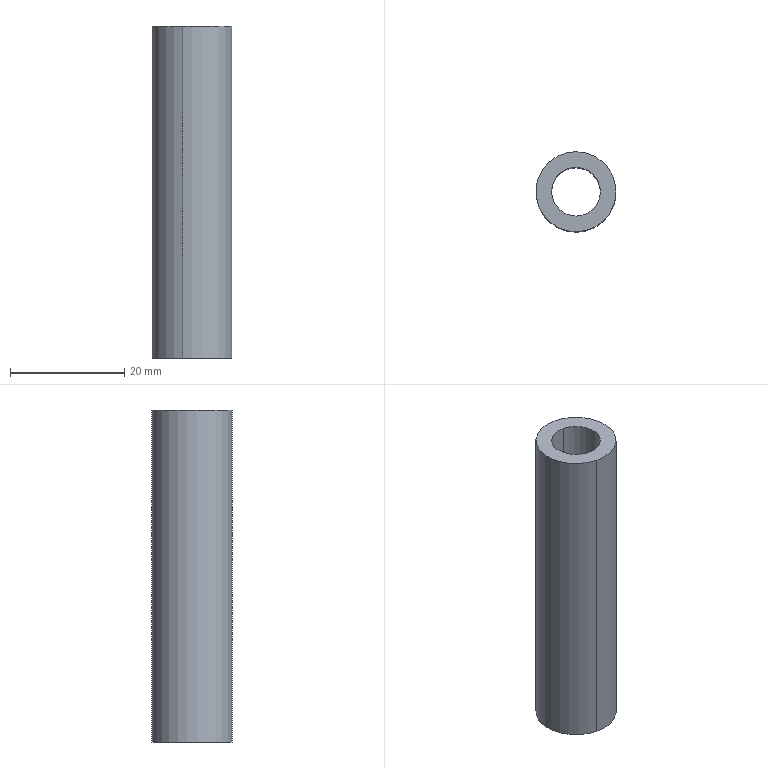Component | SolidWorks | JF21-110.2-20-1-SOLID1-1 | 1 solid | 6 faces | box 14 x 14 x 58 mm | volume 5637 mm3 | cylinder 4 | plane 2 | commonest cylinder face diameters 8.5 x2 14 x2
STEP:
#1=CARTESIAN_POINT('',(-0.03911,-0.1725,-10.984));
#2=VERTEX_POINT('',#1);
#3=CARTESIAN_POINT('',(0.03911,0.1528,-10.984));
#4=VERTEX_POINT('',#3);
#5=CARTESIAN_POINT('',(-0.,-0.009843,-10.984));
#6=DIRECTION('',(0.,-0.,1.));
#7=DIRECTION('',(0.2337,0.9723,0.));
#8=AXIS2_PLACEMENT_3D('',#5,#6,#7);
#9=CIRCLE('',#8,0.1673);
#10=EDGE_CURVE('',#2,#4,#9,.T.);
#11=ORIENTED_EDGE('',*,*,#10,.T.);
#12=CARTESIAN_POINT('',(0.03911,0.1528,-13.268));
#13=VERTEX_POINT('',#12);
#14=CARTESIAN_POINT('',(0.03911,0.1528,-10.984));
#15=DIRECTION('',(0.,-0.,1.));
#16=VECTOR('',#15,39.37);
#17=LINE('',#14,#16);
#18=EDGE_CURVE('',#13,#4,#17,.T.);
#19=ORIENTED_EDGE('',*,*,#18,.F.);
#20=CARTESIAN_POINT('',(-0.03911,-0.1725,-13.268));
#21=VERTEX_POINT('',#20);
#22=CARTESIAN_POINT('',(-0.,-0.009843,-13.268));
#23=DIRECTION('',(0.,-0.,1.));
#24=DIRECTION('',(0.2337,0.9723,0.));
#25=AXIS2_PLACEMENT_3D('',#22,#23,#24);
#26=CIRCLE('',#25,0.1673);
#27=EDGE_CURVE('',#21,#13,#26,.T.);
#28=ORIENTED_EDGE('',*,*,#27,.F.);
#29=CARTESIAN_POINT('',(-0.03911,-0.1725,-10.984));
#30=DIRECTION('',(0.,-0.,1.));
#31=VECTOR('',#30,39.37);
#32=LINE('',#29,#31);
#33=EDGE_CURVE('',#21,#2,#32,.T.);
#34=ORIENTED_EDGE('',*,*,#33,.T.);
#35=EDGE_LOOP('',(#11,#19,#28,#34));
#36=FACE_OUTER_BOUND('',#35,.T.);
#37=CARTESIAN_POINT('',(-0.,-0.009843,-10.984));
#38=DIRECTION('',(-0.,0.,-1.));
#39=DIRECTION('',(0.2337,0.9723,0.));
#40=AXIS2_PLACEMENT_3D('',#37,#38,#39);
#41=CYLINDRICAL_SURFACE('',#40,0.1673);
#42=ADVANCED_FACE('',(#36),#41,.F.);
#43=CARTESIAN_POINT('',(0.06441,0.2581,-10.984));
#44=VERTEX_POINT('',#43);
#45=CARTESIAN_POINT('',(-0.06441,-0.2778,-10.984));
#46=VERTEX_POINT('',#45);
#47=CARTESIAN_POINT('',(-0.,-0.009843,-10.984));
#48=DIRECTION('',(0.,-0.,1.));
#49=DIRECTION('',(0.2337,0.9723,0.));
#50=AXIS2_PLACEMENT_3D('',#47,#48,#49);
#51=CIRCLE('',#50,0.2756);
#52=EDGE_CURVE('',#44,#46,#51,.T.);
#53=ORIENTED_EDGE('',*,*,#52,.F.);
#54=CARTESIAN_POINT('',(0.06441,0.2581,-13.268));
#55=VERTEX_POINT('',#54);
#56=CARTESIAN_POINT('',(0.06441,0.2581,-10.984));
#57=DIRECTION('',(0.,-0.,1.));
#58=VECTOR('',#57,39.37);
#59=LINE('',#56,#58);
#60=EDGE_CURVE('',#55,#44,#59,.T.);
#61=ORIENTED_EDGE('',*,*,#60,.F.);
#62=CARTESIAN_POINT('',(-0.06441,-0.2778,-13.268));
#63=VERTEX_POINT('',#62);
#64=CARTESIAN_POINT('',(-0.,-0.009843,-13.268));
#65=DIRECTION('',(0.,-0.,1.));
#66=DIRECTION('',(0.2337,0.9723,0.));
#67=AXIS2_PLACEMENT_3D('',#64,#65,#66);
#68=CIRCLE('',#67,0.2756);
#69=EDGE_CURVE('',#55,#63,#68,.T.);
#70=ORIENTED_EDGE('',*,*,#69,.T.);
#71=CARTESIAN_POINT('',(-0.06441,-0.2778,-10.984));
#72=DIRECTION('',(0.,-0.,1.));
#73=VECTOR('',#72,39.37);
#74=LINE('',#71,#73);
#75=EDGE_CURVE('',#63,#46,#74,.T.);
#76=ORIENTED_EDGE('',*,*,#75,.T.);
#77=EDGE_LOOP('',(#53,#61,#70,#76));
#78=FACE_OUTER_BOUND('',#77,.T.);
#79=CARTESIAN_POINT('',(-0.,-0.009843,-10.984));
#80=DIRECTION('',(-0.,0.,-1.));
#81=DIRECTION('',(0.2337,0.9723,0.));
#82=AXIS2_PLACEMENT_3D('',#79,#80,#81);
#83=CYLINDRICAL_SURFACE('',#82,0.2756);
#84=ADVANCED_FACE('',(#78),#83,.T.);
#85=CARTESIAN_POINT('',(-0.,-0.009843,-10.984));
#86=DIRECTION('',(0.,-0.,1.));
#87=DIRECTION('',(0.2337,0.9723,0.));
#88=AXIS2_PLACEMENT_3D('',#85,#86,#87);
#89=CIRCLE('',#88,0.2756);
#90=EDGE_CURVE('',#46,#44,#89,.T.);
#91=ORIENTED_EDGE('',*,*,#90,.T.);
#92=ORIENTED_EDGE('',*,*,#52,.T.);
#93=EDGE_LOOP('',(#91,#92));
#94=FACE_OUTER_BOUND('',#93,.T.);
#95=ORIENTED_EDGE('',*,*,#10,.F.);
#96=CARTESIAN_POINT('',(-0.,-0.009843,-10.984));
#97=DIRECTION('',(0.,-0.,1.));
#98=DIRECTION('',(0.2337,0.9723,0.));
#99=AXIS2_PLACEMENT_3D('',#96,#97,#98);
#100=CIRCLE('',#99,0.1673);
#101=EDGE_CURVE('',#4,#2,#100,.T.);
#102=ORIENTED_EDGE('',*,*,#101,.F.);
#103=EDGE_LOOP('',(#95,#102));
#104=FACE_BOUND('',#103,.T.);
#105=CARTESIAN_POINT('',(-0.,-0.009843,-10.984));
#106=DIRECTION('',(0.,-0.,1.));
#107=DIRECTION('',(-0.2337,-0.9723,-0.));
#108=AXIS2_PLACEMENT_3D('',#105,#106,#107);
#109=PLANE('',#108);
#110=ADVANCED_FACE('',(#94,#104),#109,.T.);
#111=CARTESIAN_POINT('',(-0.,-0.009843,-13.268));
#112=DIRECTION('',(0.,-0.,1.));
#113=DIRECTION('',(0.2337,0.9723,0.));
#114=AXIS2_PLACEMENT_3D('',#111,#112,#113);
#115=CIRCLE('',#114,0.2756);
#116=EDGE_CURVE('',#63,#55,#115,.T.);
#117=ORIENTED_EDGE('',*,*,#116,.F.);
#118=ORIENTED_EDGE('',*,*,#69,.F.);
#119=EDGE_LOOP('',(#117,#118));
#120=FACE_OUTER_BOUND('',#119,.T.);
#121=ORIENTED_EDGE('',*,*,#27,.T.);
#122=CARTESIAN_POINT('',(-0.,-0.009843,-13.268));
#123=DIRECTION('',(0.,-0.,1.));
#124=DIRECTION('',(0.2337,0.9723,0.));
#125=AXIS2_PLACEMENT_3D('',#122,#123,#124);
#126=CIRCLE('',#125,0.1673);
#127=EDGE_CURVE('',#13,#21,#126,.T.);
#128=ORIENTED_EDGE('',*,*,#127,.T.);
#129=EDGE_LOOP('',(#121,#128));
#130=FACE_BOUND('',#129,.T.);
#131=CARTESIAN_POINT('',(-0.,-0.009843,-13.268));
#132=DIRECTION('',(0.,-0.,1.));
#133=DIRECTION('',(-0.2337,-0.9723,-0.));
#134=AXIS2_PLACEMENT_3D('',#131,#132,#133);
#135=PLANE('',#134);
#136=ADVANCED_FACE('',(#120,#130),#135,.F.);
#137=ORIENTED_EDGE('',*,*,#60,.T.);
#138=ORIENTED_EDGE('',*,*,#90,.F.);
#139=ORIENTED_EDGE('',*,*,#75,.F.);
#140=ORIENTED_EDGE('',*,*,#116,.T.);
#141=EDGE_LOOP('',(#137,#138,#139,#140));
#142=FACE_OUTER_BOUND('',#141,.T.);
#143=CARTESIAN_POINT('',(-0.,-0.009843,-10.984));
#144=DIRECTION('',(-0.,0.,-1.));
#145=DIRECTION('',(0.2337,0.9723,0.));
#146=AXIS2_PLACEMENT_3D('',#143,#144,#145);
#147=CYLINDRICAL_SURFACE('',#146,0.2756);
#148=ADVANCED_FACE('',(#142),#147,.T.);
#149=ORIENTED_EDGE('',*,*,#18,.T.);
#150=ORIENTED_EDGE('',*,*,#101,.T.);
#151=ORIENTED_EDGE('',*,*,#33,.F.);
#152=ORIENTED_EDGE('',*,*,#127,.F.);
#153=EDGE_LOOP('',(#149,#150,#151,#152));
#154=FACE_OUTER_BOUND('',#153,.T.);
#155=CARTESIAN_POINT('',(-0.,-0.009843,-10.984));
#156=DIRECTION('',(-0.,0.,-1.));
#157=DIRECTION('',(0.2337,0.9723,0.));
#158=AXIS2_PLACEMENT_3D('',#155,#156,#157);
#159=CYLINDRICAL_SURFACE('',#158,0.1673);
#160=ADVANCED_FACE('',(#154),#159,.F.);
#161=CLOSED_SHELL('',(#42,#84,#110,#136,#148,#160));
#162=MANIFOLD_SOLID_BREP('',#161);
#163=CARTESIAN_POINT('',(0.,0.,0.));
#164=DIRECTION('',(0.,0.,1.));
#165=DIRECTION('',(1.,0.,0.));
#166=AXIS2_PLACEMENT_3D('',#163,#164,#165);
#167=(LENGTH_UNIT()NAMED_UNIT(*)SI_UNIT($,.METRE.));
#168=LENGTH_MEASURE_WITH_UNIT(LENGTH_MEASURE(0.0254),#167);
#169=DIMENSIONAL_EXPONENTS(1.,0.,0.,0.,0.,0.,0.);
#170=(CONVERSION_BASED_UNIT('',#168)LENGTH_UNIT()NAMED_UNIT(#169));
#171=UNCERTAINTY_MEASURE_WITH_UNIT(LENGTH_MEASURE(0.00001),#170,'','');
#172=(NAMED_UNIT(*)PLANE_ANGLE_UNIT()SI_UNIT($,.RADIAN.));
#173=(NAMED_UNIT(*)SI_UNIT($,.STERADIAN.)SOLID_ANGLE_UNIT());
#174=(GEOMETRIC_REPRESENTATION_CONTEXT(3)GLOBAL_UNCERTAINTY_ASSIGNED_CONTEXT((#171))GLOBAL_UNIT_ASSIGNED_CONTEXT((#170,#172,#173))REPRESENTATION_CONTEXT('',''));
#175=ADVANCED_BREP_SHAPE_REPRESENTATION('',(#162,#166),#174);
#176=COLOUR_RGB('',0.7922,0.8196,0.9333);
#177=FILL_AREA_STYLE_COLOUR('',#176);
#178=FILL_AREA_STYLE('',(#177));
#179=SURFACE_STYLE_FILL_AREA(#178);
#180=SURFACE_SIDE_STYLE('',(#179));
#181=SURFACE_STYLE_USAGE(.BOTH.,#180);
#182=PRESENTATION_STYLE_ASSIGNMENT((#181));
#183=STYLED_ITEM('',(#182),#162);
#184=PRESENTATION_LAYER_ASSIGNMENT('','',(#183));
#185=(LENGTH_UNIT()NAMED_UNIT(*)SI_UNIT($,.METRE.));
#186=LENGTH_MEASURE_WITH_UNIT(LENGTH_MEASURE(0.0254),#185);
#187=DIMENSIONAL_EXPONENTS(1.,0.,0.,0.,0.,0.,0.);
#188=(CONVERSION_BASED_UNIT('',#186)LENGTH_UNIT()NAMED_UNIT(#187));
#189=UNCERTAINTY_MEASURE_WITH_UNIT(LENGTH_MEASURE(0.00001),#188,'','');
#190=(NAMED_UNIT(*)PLANE_ANGLE_UNIT()SI_UNIT($,.RADIAN.));
#191=(NAMED_UNIT(*)SI_UNIT($,.STERADIAN.)SOLID_ANGLE_UNIT());
#192=(GEOMETRIC_REPRESENTATION_CONTEXT(3)GLOBAL_UNCERTAINTY_ASSIGNED_CONTEXT((#189))GLOBAL_UNIT_ASSIGNED_CONTEXT((#188,#190,#191))REPRESENTATION_CONTEXT('',''));
#193=MECHANICAL_DESIGN_GEOMETRIC_PRESENTATION_REPRESENTATION('',(#183),#192);